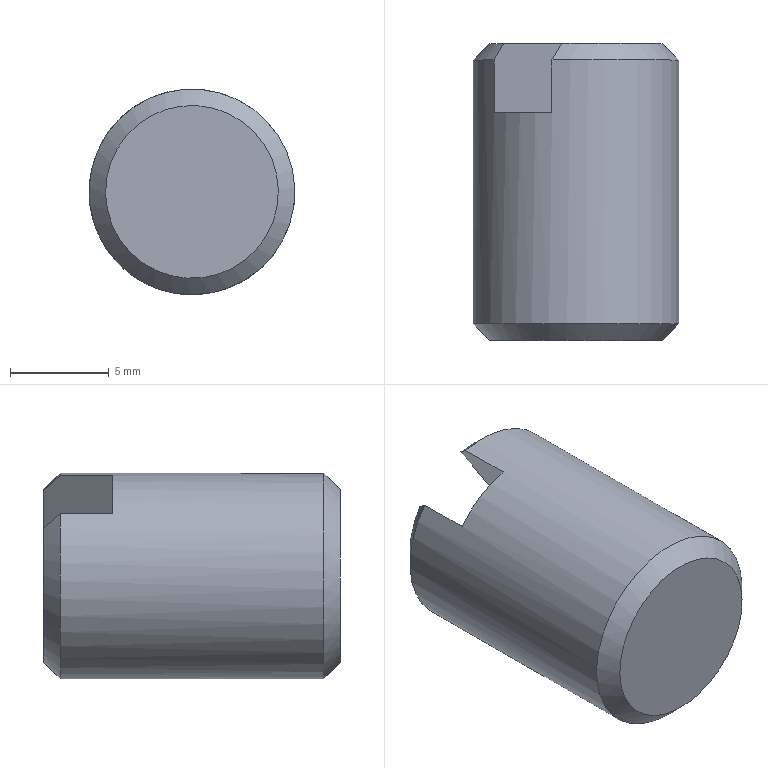Component | NX | 12_PRESSURE_PIN | 1 solid | 10 faces | box 10.4 x 15 x 10.4 mm | volume 1129 mm3 | plane 6 | cone 3 | cylinder 1 | commonest cylinder face diameters 10.396 x1
STEP:
#1=CARTESIAN_POINT('',(0.,0.,0.));
#2=DIRECTION('',(0.,0.,1.));
#3=DIRECTION('',(1.,0.,0.));
#4=AXIS2_PLACEMENT_3D('',#1,#2,#3);
#5=CARTESIAN_POINT('',(-55.431,208.794,-240.61));
#6=VERTEX_POINT('',#5);
#7=CARTESIAN_POINT('',(-59.806,208.794,-233.913));
#8=VERTEX_POINT('',#7);
#9=CARTESIAN_POINT('',(-57.619,208.794,-237.262));
#10=DIRECTION('',(-0.5469,0.,0.8372));
#11=VECTOR('',#10,1.);
#12=LINE('',#9,#11);
#13=CARTESIAN_POINT('',(-59.084,208.794,-238.219));
#14=DIRECTION('',(0.,1.,0.));
#15=DIRECTION('',(0.8372,0.,0.5469));
#16=AXIS2_PLACEMENT_3D('',#13,#14,#15);
#17=PLANE('',#16);
#18=CARTESIAN_POINT('',(1.75,0.));
#19=DIRECTION('',(0.,-1.));
#20=VECTOR('',#19,1.);
#21=LINE('',#18,#20);
#22=(GEOMETRIC_REPRESENTATION_CONTEXT(2)PARAMETRIC_REPRESENTATION_CONTEXT()REPRESENTATION_CONTEXT('',''));
#23=DEFINITIONAL_REPRESENTATION('',(#21),#22);
#24=PCURVE('',#17,#23);
#25=CARTESIAN_POINT('',(-54.337,205.294,-242.285));
#26=DIRECTION('',(-0.8372,0.,-0.5469));
#27=DIRECTION('',(-0.5469,0.,0.8372));
#28=AXIS2_PLACEMENT_3D('',#25,#26,#27);
#29=PLANE('',#28);
#30=CARTESIAN_POINT('',(6.,3.5));
#31=DIRECTION('',(1.,0.));
#32=VECTOR('',#31,1.);
#33=LINE('',#30,#32);
#34=(GEOMETRIC_REPRESENTATION_CONTEXT(2)PARAMETRIC_REPRESENTATION_CONTEXT()REPRESENTATION_CONTEXT('',''));
#35=DEFINITIONAL_REPRESENTATION('',(#33),#34);
#36=PCURVE('',#29,#35);
#37=SURFACE_CURVE('',#12,(#24,#36),.PCURVE_S1.);
#38=EDGE_CURVE('',#6,#8,#37,.T.);
#39=ORIENTED_EDGE('',*,*,#38,.T.);
#40=CARTESIAN_POINT('',(-59.084,208.794,-238.219));
#41=DIRECTION('',(0.,1.,0.));
#42=DIRECTION('',(0.8372,0.,0.5469));
#43=AXIS2_PLACEMENT_3D('',#40,#41,#42);
#44=CIRCLE('',#43,4.366);
#45=CARTESIAN_POINT('',(0.,0.));
#46=DIRECTION('',(1.,-0.));
#47=AXIS2_PLACEMENT_2D('',#45,#46);
#48=CIRCLE('',#47,4.366);
#49=(GEOMETRIC_REPRESENTATION_CONTEXT(2)PARAMETRIC_REPRESENTATION_CONTEXT()REPRESENTATION_CONTEXT('',''));
#50=DEFINITIONAL_REPRESENTATION('',(#48),#49);
#51=PCURVE('',#17,#50);
#52=CARTESIAN_POINT('',(-59.084,207.727,-238.219));
#53=DIRECTION('',(0.,-1.,0.));
#54=DIRECTION('',(-0.8372,0.,-0.5469));
#55=AXIS2_PLACEMENT_3D('',#52,#53,#54);
#56=CONICAL_SURFACE('',#55,5.433,0.7854);
#57=CARTESIAN_POINT('',(9.425,-1.067));
#58=DIRECTION('',(-1.,0.));
#59=VECTOR('',#58,1.);
#60=LINE('',#57,#59);
#61=(GEOMETRIC_REPRESENTATION_CONTEXT(2)PARAMETRIC_REPRESENTATION_CONTEXT()REPRESENTATION_CONTEXT('',''));
#62=DEFINITIONAL_REPRESENTATION('',(#60),#61);
#63=PCURVE('',#56,#62);
#64=SURFACE_CURVE('',#44,(#51,#63),.PCURVE_S1.);
#65=EDGE_CURVE('',#8,#6,#64,.T.);
#66=ORIENTED_EDGE('',*,*,#65,.T.);
#67=EDGE_LOOP('',(#39,#66));
#68=FACE_BOUND('',#67,.T.);
#69=ADVANCED_FACE('',(#68),#17,.T.);
#70=CARTESIAN_POINT('',(-58.361,208.794,-242.525));
#71=VERTEX_POINT('',#70);
#72=CARTESIAN_POINT('',(-62.736,208.794,-235.828));
#73=VERTEX_POINT('',#72);
#74=CARTESIAN_POINT('',(-60.549,208.794,-239.176));
#75=DIRECTION('',(-0.5469,0.,0.8372));
#76=VECTOR('',#75,1.);
#77=LINE('',#74,#76);
#78=CARTESIAN_POINT('',(-59.084,208.794,-238.219));
#79=DIRECTION('',(0.,1.,0.));
#80=DIRECTION('',(0.8372,0.,0.5469));
#81=AXIS2_PLACEMENT_3D('',#78,#79,#80);
#82=PLANE('',#81);
#83=CARTESIAN_POINT('',(-1.75,0.));
#84=DIRECTION('',(0.,-1.));
#85=VECTOR('',#84,1.);
#86=LINE('',#83,#85);
#87=(GEOMETRIC_REPRESENTATION_CONTEXT(2)PARAMETRIC_REPRESENTATION_CONTEXT()REPRESENTATION_CONTEXT('',''));
#88=DEFINITIONAL_REPRESENTATION('',(#86),#87);
#89=PCURVE('',#82,#88);
#90=CARTESIAN_POINT('',(-57.267,205.294,-244.199));
#91=DIRECTION('',(-0.8372,0.,-0.5469));
#92=DIRECTION('',(-0.5469,0.,0.8372));
#93=AXIS2_PLACEMENT_3D('',#90,#91,#92);
#94=PLANE('',#93);
#95=CARTESIAN_POINT('',(6.,3.5));
#96=DIRECTION('',(1.,0.));
#97=VECTOR('',#96,1.);
#98=LINE('',#95,#97);
#99=(GEOMETRIC_REPRESENTATION_CONTEXT(2)PARAMETRIC_REPRESENTATION_CONTEXT()REPRESENTATION_CONTEXT('',''));
#100=DEFINITIONAL_REPRESENTATION('',(#98),#99);
#101=PCURVE('',#94,#100);
#102=SURFACE_CURVE('',#77,(#89,#101),.PCURVE_S1.);
#103=EDGE_CURVE('',#71,#73,#102,.T.);
#104=ORIENTED_EDGE('',*,*,#103,.F.);
#105=CARTESIAN_POINT('',(-59.084,208.794,-238.219));
#106=DIRECTION('',(0.,1.,0.));
#107=DIRECTION('',(0.8372,0.,0.5469));
#108=AXIS2_PLACEMENT_3D('',#105,#106,#107);
#109=CIRCLE('',#108,4.366);
#110=CARTESIAN_POINT('',(0.,0.));
#111=DIRECTION('',(1.,-0.));
#112=AXIS2_PLACEMENT_2D('',#110,#111);
#113=CIRCLE('',#112,4.366);
#114=(GEOMETRIC_REPRESENTATION_CONTEXT(2)PARAMETRIC_REPRESENTATION_CONTEXT()REPRESENTATION_CONTEXT('',''));
#115=DEFINITIONAL_REPRESENTATION('',(#113),#114);
#116=PCURVE('',#82,#115);
#117=CARTESIAN_POINT('',(-59.084,207.727,-238.219));
#118=DIRECTION('',(0.,-1.,0.));
#119=DIRECTION('',(-0.8372,0.,-0.5469));
#120=AXIS2_PLACEMENT_3D('',#117,#118,#119);
#121=CONICAL_SURFACE('',#120,5.433,0.7854);
#122=CARTESIAN_POINT('',(3.142,-1.067));
#123=DIRECTION('',(-1.,-0.));
#124=VECTOR('',#123,1.);
#125=LINE('',#122,#124);
#126=(GEOMETRIC_REPRESENTATION_CONTEXT(2)PARAMETRIC_REPRESENTATION_CONTEXT()REPRESENTATION_CONTEXT('',''));
#127=DEFINITIONAL_REPRESENTATION('',(#125),#126);
#128=PCURVE('',#121,#127);
#129=SURFACE_CURVE('',#109,(#116,#128),.PCURVE_S1.);
#130=EDGE_CURVE('',#71,#73,#129,.T.);
#131=ORIENTED_EDGE('',*,*,#130,.T.);
#132=EDGE_LOOP('',(#104,#131));
#133=FACE_BOUND('',#132,.T.);
#134=ADVANCED_FACE('',(#133),#82,.T.);
#135=CARTESIAN_POINT('',(-62.739,193.794,-240.607));
#136=VERTEX_POINT('',#135);
#137=CARTESIAN_POINT('',(-55.429,193.794,-235.831));
#138=VERTEX_POINT('',#137);
#139=CARTESIAN_POINT('',(-59.084,193.794,-238.219));
#140=DIRECTION('',(0.,-1.,0.));
#141=DIRECTION('',(-0.8372,0.,-0.5469));
#142=AXIS2_PLACEMENT_3D('',#139,#140,#141);
#143=CIRCLE('',#142,4.366);
#144=CARTESIAN_POINT('',(-59.084,193.794,-238.219));
#145=DIRECTION('',(0.,-1.,0.));
#146=DIRECTION('',(-0.8372,0.,-0.5469));
#147=AXIS2_PLACEMENT_3D('',#144,#145,#146);
#148=PLANE('',#147);
#149=CARTESIAN_POINT('',(0.,0.));
#150=DIRECTION('',(1.,0.));
#151=AXIS2_PLACEMENT_2D('',#149,#150);
#152=CIRCLE('',#151,4.366);
#153=(GEOMETRIC_REPRESENTATION_CONTEXT(2)PARAMETRIC_REPRESENTATION_CONTEXT()REPRESENTATION_CONTEXT('',''));
#154=DEFINITIONAL_REPRESENTATION('',(#152),#153);
#155=PCURVE('',#148,#154);
#156=CARTESIAN_POINT('',(-59.084,194.861,-238.219));
#157=DIRECTION('',(0.,1.,0.));
#158=DIRECTION('',(0.8372,0.,0.5469));
#159=AXIS2_PLACEMENT_3D('',#156,#157,#158);
#160=CONICAL_SURFACE('',#159,5.433,0.7854);
#161=CARTESIAN_POINT('',(3.142,-1.067));
#162=DIRECTION('',(-1.,0.));
#163=VECTOR('',#162,1.);
#164=LINE('',#161,#163);
#165=(GEOMETRIC_REPRESENTATION_CONTEXT(2)PARAMETRIC_REPRESENTATION_CONTEXT()REPRESENTATION_CONTEXT('',''));
#166=DEFINITIONAL_REPRESENTATION('',(#164),#165);
#167=PCURVE('',#160,#166);
#168=SURFACE_CURVE('',#143,(#155,#167),.PCURVE_S1.);
#169=EDGE_CURVE('',#136,#138,#168,.T.);
#170=ORIENTED_EDGE('',*,*,#169,.T.);
#171=CARTESIAN_POINT('',(-59.084,193.794,-238.219));
#172=DIRECTION('',(0.,-1.,0.));
#173=DIRECTION('',(-0.8372,0.,-0.5469));
#174=AXIS2_PLACEMENT_3D('',#171,#172,#173);
#175=CIRCLE('',#174,4.366);
#176=CARTESIAN_POINT('',(0.,0.));
#177=DIRECTION('',(1.,0.));
#178=AXIS2_PLACEMENT_2D('',#176,#177);
#179=CIRCLE('',#178,4.366);
#180=(GEOMETRIC_REPRESENTATION_CONTEXT(2)PARAMETRIC_REPRESENTATION_CONTEXT()REPRESENTATION_CONTEXT('',''));
#181=DEFINITIONAL_REPRESENTATION('',(#179),#180);
#182=PCURVE('',#148,#181);
#183=CARTESIAN_POINT('',(9.425,-1.067));
#184=DIRECTION('',(-1.,0.));
#185=VECTOR('',#184,1.);
#186=LINE('',#183,#185);
#187=(GEOMETRIC_REPRESENTATION_CONTEXT(2)PARAMETRIC_REPRESENTATION_CONTEXT()REPRESENTATION_CONTEXT('',''));
#188=DEFINITIONAL_REPRESENTATION('',(#186),#187);
#189=PCURVE('',#160,#188);
#190=SURFACE_CURVE('',#175,(#182,#189),.PCURVE_S1.);
#191=EDGE_CURVE('',#138,#136,#190,.T.);
#192=ORIENTED_EDGE('',*,*,#191,.T.);
#193=EDGE_LOOP('',(#170,#192));
#194=FACE_BOUND('',#193,.T.);
#195=ADVANCED_FACE('',(#194),#148,.T.);
#196=CARTESIAN_POINT('',(-54.732,194.626,-235.376));
#197=VERTEX_POINT('',#196);
#198=CARTESIAN_POINT('',(-59.084,194.626,-238.219));
#199=DIRECTION('',(0.,1.,0.));
#200=DIRECTION('',(0.8372,0.,0.5469));
#201=AXIS2_PLACEMENT_3D('',#198,#199,#200);
#202=CIRCLE('',#201,5.198);
#203=CARTESIAN_POINT('',(-59.084,193.794,-238.219));
#204=DIRECTION('',(0.,1.,0.));
#205=DIRECTION('',(0.8372,0.,0.5469));
#206=AXIS2_PLACEMENT_3D('',#203,#204,#205);
#207=CYLINDRICAL_SURFACE('',#206,5.198);
#208=CARTESIAN_POINT('',(0.,0.8322));
#209=DIRECTION('',(1.,0.));
#210=VECTOR('',#209,1.);
#211=LINE('',#208,#210);
#212=(GEOMETRIC_REPRESENTATION_CONTEXT(2)PARAMETRIC_REPRESENTATION_CONTEXT()REPRESENTATION_CONTEXT('',''));
#213=DEFINITIONAL_REPRESENTATION('',(#211),#212);
#214=PCURVE('',#207,#213);
#215=CARTESIAN_POINT('',(0.,-0.2349));
#216=DIRECTION('',(1.,0.));
#217=VECTOR('',#216,1.);
#218=LINE('',#215,#217);
#219=(GEOMETRIC_REPRESENTATION_CONTEXT(2)PARAMETRIC_REPRESENTATION_CONTEXT()REPRESENTATION_CONTEXT('',''));
#220=DEFINITIONAL_REPRESENTATION('',(#218),#219);
#221=PCURVE('',#160,#220);
#222=SURFACE_CURVE('',#202,(#214,#221),.PCURVE_S1.);
#223=EDGE_CURVE('',#197,#197,#222,.T.);
#224=ORIENTED_EDGE('',*,*,#223,.T.);
#225=CARTESIAN_POINT('',(-54.732,207.961,-235.376));
#226=VERTEX_POINT('',#225);
#227=CARTESIAN_POINT('',(-54.732,194.626,-235.376));
#228=CARTESIAN_POINT('',(-54.732,207.961,-235.376));
#229=B_SPLINE_CURVE_WITH_KNOTS('',1,(#227,#228),.UNSPECIFIED.,.F.,.F.,(2,2),(0.8322,14.168),.PIECEWISE_BEZIER_KNOTS.);
#230=CARTESIAN_POINT('',(6.283,0.));
#231=DIRECTION('',(0.,1.));
#232=VECTOR('',#231,1.);
#233=LINE('',#230,#232);
#234=(GEOMETRIC_REPRESENTATION_CONTEXT(2)PARAMETRIC_REPRESENTATION_CONTEXT()REPRESENTATION_CONTEXT('',''));
#235=DEFINITIONAL_REPRESENTATION('',(#233),#234);
#236=PCURVE('',#207,#235);
#237=CARTESIAN_POINT('',(0.,0.));
#238=DIRECTION('',(0.,1.));
#239=VECTOR('',#238,1.);
#240=LINE('',#237,#239);
#241=(GEOMETRIC_REPRESENTATION_CONTEXT(2)PARAMETRIC_REPRESENTATION_CONTEXT()REPRESENTATION_CONTEXT('',''));
#242=DEFINITIONAL_REPRESENTATION('',(#240),#241);
#243=PCURVE('',#207,#242);
#244=SEAM_CURVE('',#229,(#236,#243),.PCURVE_S1.);
#245=EDGE_CURVE('',#197,#226,#244,.T.);
#246=ORIENTED_EDGE('',*,*,#245,.T.);
#247=CARTESIAN_POINT('',(-60.296,207.961,-233.164));
#248=VERTEX_POINT('',#247);
#249=CARTESIAN_POINT('',(-59.084,207.961,-238.219));
#250=DIRECTION('',(0.,-1.,0.));
#251=DIRECTION('',(-0.8372,0.,-0.5469));
#252=AXIS2_PLACEMENT_3D('',#249,#250,#251);
#253=CIRCLE('',#252,5.198);
#254=CARTESIAN_POINT('',(9.425,14.168));
#255=DIRECTION('',(-1.,0.));
#256=VECTOR('',#255,1.);
#257=LINE('',#254,#256);
#258=(GEOMETRIC_REPRESENTATION_CONTEXT(2)PARAMETRIC_REPRESENTATION_CONTEXT()REPRESENTATION_CONTEXT('',''));
#259=DEFINITIONAL_REPRESENTATION('',(#257),#258);
#260=PCURVE('',#207,#259);
#261=CARTESIAN_POINT('',(-0.,-0.2349));
#262=DIRECTION('',(1.,-0.));
#263=VECTOR('',#262,1.);
#264=LINE('',#261,#263);
#265=(GEOMETRIC_REPRESENTATION_CONTEXT(2)PARAMETRIC_REPRESENTATION_CONTEXT()REPRESENTATION_CONTEXT('',''));
#266=DEFINITIONAL_REPRESENTATION('',(#264),#265);
#267=PCURVE('',#56,#266);
#268=SURFACE_CURVE('',#253,(#260,#267),.PCURVE_S1.);
#269=EDGE_CURVE('',#226,#248,#268,.T.);
#270=ORIENTED_EDGE('',*,*,#269,.T.);
#271=CARTESIAN_POINT('',(-60.296,205.294,-233.164));
#272=VERTEX_POINT('',#271);
#273=CARTESIAN_POINT('',(-60.296,207.961,-233.164));
#274=DIRECTION('',(0.,-1.,0.));
#275=VECTOR('',#274,1.);
#276=LINE('',#273,#275);
#277=CARTESIAN_POINT('',(5.056,14.168));
#278=DIRECTION('',(0.,-1.));
#279=VECTOR('',#278,1.);
#280=LINE('',#277,#279);
#281=(GEOMETRIC_REPRESENTATION_CONTEXT(2)PARAMETRIC_REPRESENTATION_CONTEXT()REPRESENTATION_CONTEXT('',''));
#282=DEFINITIONAL_REPRESENTATION('',(#280),#281);
#283=PCURVE('',#207,#282);
#284=CARTESIAN_POINT('',(10.895,2.668));
#285=DIRECTION('',(0.,-1.));
#286=VECTOR('',#285,1.);
#287=LINE('',#284,#286);
#288=(GEOMETRIC_REPRESENTATION_CONTEXT(2)PARAMETRIC_REPRESENTATION_CONTEXT()REPRESENTATION_CONTEXT('',''));
#289=DEFINITIONAL_REPRESENTATION('',(#287),#288);
#290=PCURVE('',#29,#289);
#291=SURFACE_CURVE('',#276,(#283,#290),.PCURVE_S1.);
#292=EDGE_CURVE('',#248,#272,#291,.T.);
#293=ORIENTED_EDGE('',*,*,#292,.T.);
#294=CARTESIAN_POINT('',(-63.226,205.294,-235.079));
#295=VERTEX_POINT('',#294);
#296=CARTESIAN_POINT('',(-59.084,205.294,-238.219));
#297=DIRECTION('',(0.,1.,0.));
#298=DIRECTION('',(-0.8372,0.,-0.5469));
#299=AXIS2_PLACEMENT_3D('',#296,#297,#298);
#300=CIRCLE('',#299,5.198);
#301=CARTESIAN_POINT('',(3.142,11.5));
#302=DIRECTION('',(1.,0.));
#303=VECTOR('',#302,1.);
#304=LINE('',#301,#303);
#305=(GEOMETRIC_REPRESENTATION_CONTEXT(2)PARAMETRIC_REPRESENTATION_CONTEXT()REPRESENTATION_CONTEXT('',''));
#306=DEFINITIONAL_REPRESENTATION('',(#304),#305);
#307=PCURVE('',#207,#306);
#308=CARTESIAN_POINT('',(-55.802,205.294,-243.242));
#309=DIRECTION('',(0.,-1.,0.));
#310=DIRECTION('',(-0.5469,0.,0.8372));
#311=AXIS2_PLACEMENT_3D('',#308,#309,#310);
#312=PLANE('',#311);
#313=CARTESIAN_POINT('',(6.,5.198));
#314=CARTESIAN_POINT('',(15.003,5.198));
#315=CARTESIAN_POINT('',(10.502,-2.599));
#316=CARTESIAN_POINT('',(6.,-10.396));
#317=CARTESIAN_POINT('',(1.498,-2.599));
#318=CARTESIAN_POINT('',(-3.003,5.198));
#319=CARTESIAN_POINT('',(6.,5.198));
#320=(BOUNDED_CURVE()B_SPLINE_CURVE(2,(#313,#314,#315,#316,#317,#318,#319),.UNSPECIFIED.,.T.,.F.)B_SPLINE_CURVE_WITH_KNOTS((1,2,2,2,2,1),(-2.094,0.,2.094,4.189,6.283,8.378),.UNSPECIFIED.)CURVE()GEOMETRIC_REPRESENTATION_ITEM()RATIONAL_B_SPLINE_CURVE((1.,0.5,1.,0.5,1.,0.5,1.))REPRESENTATION_ITEM(''));
#321=(GEOMETRIC_REPRESENTATION_CONTEXT(2)PARAMETRIC_REPRESENTATION_CONTEXT()REPRESENTATION_CONTEXT('',''));
#322=DEFINITIONAL_REPRESENTATION('',(#320),#321);
#323=PCURVE('',#312,#322);
#324=SURFACE_CURVE('',#300,(#307,#323),.PCURVE_S1.);
#325=EDGE_CURVE('',#295,#272,#324,.T.);
#326=ORIENTED_EDGE('',*,*,#325,.F.);
#327=CARTESIAN_POINT('',(-63.226,207.961,-235.079));
#328=VERTEX_POINT('',#327);
#329=CARTESIAN_POINT('',(-63.226,193.794,-235.079));
#330=DIRECTION('',(0.,-1.,0.));
#331=VECTOR('',#330,1.);
#332=LINE('',#329,#331);
#333=CARTESIAN_POINT('',(4.369,0.));
#334=DIRECTION('',(0.,-1.));
#335=VECTOR('',#334,1.);
#336=LINE('',#333,#335);
#337=(GEOMETRIC_REPRESENTATION_CONTEXT(2)PARAMETRIC_REPRESENTATION_CONTEXT()REPRESENTATION_CONTEXT('',''));
#338=DEFINITIONAL_REPRESENTATION('',(#336),#337);
#339=PCURVE('',#207,#338);
#340=CARTESIAN_POINT('',(10.895,-11.5));
#341=DIRECTION('',(0.,-1.));
#342=VECTOR('',#341,1.);
#343=LINE('',#340,#342);
#344=(GEOMETRIC_REPRESENTATION_CONTEXT(2)PARAMETRIC_REPRESENTATION_CONTEXT()REPRESENTATION_CONTEXT('',''));
#345=DEFINITIONAL_REPRESENTATION('',(#343),#344);
#346=PCURVE('',#94,#345);
#347=SURFACE_CURVE('',#332,(#339,#346),.PCURVE_S1.);
#348=EDGE_CURVE('',#328,#295,#347,.T.);
#349=ORIENTED_EDGE('',*,*,#348,.F.);
#350=CARTESIAN_POINT('',(-57.872,207.961,-243.274));
#351=VERTEX_POINT('',#350);
#352=CARTESIAN_POINT('',(-59.084,207.961,-238.219));
#353=DIRECTION('',(0.,-1.,0.));
#354=DIRECTION('',(-0.8372,0.,-0.5469));
#355=AXIS2_PLACEMENT_3D('',#352,#353,#354);
#356=CIRCLE('',#355,5.198);
#357=CARTESIAN_POINT('',(9.425,14.168));
#358=DIRECTION('',(-1.,0.));
#359=VECTOR('',#358,1.);
#360=LINE('',#357,#359);
#361=(GEOMETRIC_REPRESENTATION_CONTEXT(2)PARAMETRIC_REPRESENTATION_CONTEXT()REPRESENTATION_CONTEXT('',''));
#362=DEFINITIONAL_REPRESENTATION('',(#360),#361);
#363=PCURVE('',#207,#362);
#364=CARTESIAN_POINT('',(-6.283,-0.2349));
#365=DIRECTION('',(1.,0.));
#366=VECTOR('',#365,1.);
#367=LINE('',#364,#366);
#368=(GEOMETRIC_REPRESENTATION_CONTEXT(2)PARAMETRIC_REPRESENTATION_CONTEXT()REPRESENTATION_CONTEXT('',''));
#369=DEFINITIONAL_REPRESENTATION('',(#367),#368);
#370=PCURVE('',#121,#369);
#371=SURFACE_CURVE('',#356,(#363,#370),.PCURVE_S1.);
#372=EDGE_CURVE('',#328,#351,#371,.T.);
#373=ORIENTED_EDGE('',*,*,#372,.T.);
#374=CARTESIAN_POINT('',(-57.872,205.294,-243.274));
#375=VERTEX_POINT('',#374);
#376=CARTESIAN_POINT('',(-57.872,205.294,-243.274));
#377=DIRECTION('',(0.,1.,0.));
#378=VECTOR('',#377,1.);
#379=LINE('',#376,#378);
#380=CARTESIAN_POINT('',(1.914,11.5));
#381=DIRECTION('',(0.,1.));
#382=VECTOR('',#381,1.);
#383=LINE('',#380,#382);
#384=(GEOMETRIC_REPRESENTATION_CONTEXT(2)PARAMETRIC_REPRESENTATION_CONTEXT()REPRESENTATION_CONTEXT('',''));
#385=DEFINITIONAL_REPRESENTATION('',(#383),#384);
#386=PCURVE('',#207,#385);
#387=CARTESIAN_POINT('',(1.105,0.));
#388=DIRECTION('',(0.,1.));
#389=VECTOR('',#388,1.);
#390=LINE('',#387,#389);
#391=(GEOMETRIC_REPRESENTATION_CONTEXT(2)PARAMETRIC_REPRESENTATION_CONTEXT()REPRESENTATION_CONTEXT('',''));
#392=DEFINITIONAL_REPRESENTATION('',(#390),#391);
#393=PCURVE('',#94,#392);
#394=SURFACE_CURVE('',#379,(#386,#393),.PCURVE_S1.);
#395=EDGE_CURVE('',#375,#351,#394,.T.);
#396=ORIENTED_EDGE('',*,*,#395,.F.);
#397=CARTESIAN_POINT('',(-54.942,205.294,-241.359));
#398=VERTEX_POINT('',#397);
#399=CARTESIAN_POINT('',(-59.084,205.294,-238.219));
#400=DIRECTION('',(0.,1.,0.));
#401=DIRECTION('',(-0.8372,0.,-0.5469));
#402=AXIS2_PLACEMENT_3D('',#399,#400,#401);
#403=CIRCLE('',#402,5.198);
#404=CARTESIAN_POINT('',(-3.142,11.5));
#405=DIRECTION('',(1.,0.));
#406=VECTOR('',#405,1.);
#407=LINE('',#404,#406);
#408=(GEOMETRIC_REPRESENTATION_CONTEXT(2)PARAMETRIC_REPRESENTATION_CONTEXT()REPRESENTATION_CONTEXT('',''));
#409=DEFINITIONAL_REPRESENTATION('',(#407),#408);
#410=PCURVE('',#207,#409);
#411=CARTESIAN_POINT('',(6.,5.198));
#412=CARTESIAN_POINT('',(15.003,5.198));
#413=CARTESIAN_POINT('',(10.502,-2.599));
#414=CARTESIAN_POINT('',(6.,-10.396));
#415=CARTESIAN_POINT('',(1.498,-2.599));
#416=CARTESIAN_POINT('',(-3.003,5.198));
#417=CARTESIAN_POINT('',(6.,5.198));
#418=(BOUNDED_CURVE()B_SPLINE_CURVE(2,(#411,#412,#413,#414,#415,#416,#417),.UNSPECIFIED.,.T.,.F.)B_SPLINE_CURVE_WITH_KNOTS((1,2,2,2,2,1),(-2.094,0.,2.094,4.189,6.283,8.378),.UNSPECIFIED.)CURVE()GEOMETRIC_REPRESENTATION_ITEM()RATIONAL_B_SPLINE_CURVE((1.,0.5,1.,0.5,1.,0.5,1.))REPRESENTATION_ITEM(''));
#419=(GEOMETRIC_REPRESENTATION_CONTEXT(2)PARAMETRIC_REPRESENTATION_CONTEXT()REPRESENTATION_CONTEXT('',''));
#420=DEFINITIONAL_REPRESENTATION('',(#418),#419);
#421=PCURVE('',#312,#420);
#422=SURFACE_CURVE('',#403,(#410,#421),.PCURVE_S1.);
#423=EDGE_CURVE('',#398,#375,#422,.T.);
#424=ORIENTED_EDGE('',*,*,#423,.F.);
#425=CARTESIAN_POINT('',(-54.942,207.961,-241.359));
#426=VERTEX_POINT('',#425);
#427=CARTESIAN_POINT('',(-54.942,193.794,-241.359));
#428=DIRECTION('',(0.,1.,0.));
#429=VECTOR('',#428,1.);
#430=LINE('',#427,#429);
#431=CARTESIAN_POINT('',(1.227,0.));
#432=DIRECTION('',(0.,1.));
#433=VECTOR('',#432,1.);
#434=LINE('',#431,#433);
#435=(GEOMETRIC_REPRESENTATION_CONTEXT(2)PARAMETRIC_REPRESENTATION_CONTEXT()REPRESENTATION_CONTEXT('',''));
#436=DEFINITIONAL_REPRESENTATION('',(#434),#435);
#437=PCURVE('',#207,#436);
#438=CARTESIAN_POINT('',(1.105,-11.5));
#439=DIRECTION('',(0.,1.));
#440=VECTOR('',#439,1.);
#441=LINE('',#438,#440);
#442=(GEOMETRIC_REPRESENTATION_CONTEXT(2)PARAMETRIC_REPRESENTATION_CONTEXT()REPRESENTATION_CONTEXT('',''));
#443=DEFINITIONAL_REPRESENTATION('',(#441),#442);
#444=PCURVE('',#29,#443);
#445=SURFACE_CURVE('',#430,(#437,#444),.PCURVE_S1.);
#446=EDGE_CURVE('',#398,#426,#445,.T.);
#447=ORIENTED_EDGE('',*,*,#446,.T.);
#448=CARTESIAN_POINT('',(-59.084,207.961,-238.219));
#449=DIRECTION('',(0.,-1.,0.));
#450=DIRECTION('',(-0.8372,0.,-0.5469));
#451=AXIS2_PLACEMENT_3D('',#448,#449,#450);
#452=CIRCLE('',#451,5.198);
#453=CARTESIAN_POINT('',(3.142,14.168));
#454=DIRECTION('',(-1.,0.));
#455=VECTOR('',#454,1.);
#456=LINE('',#453,#455);
#457=(GEOMETRIC_REPRESENTATION_CONTEXT(2)PARAMETRIC_REPRESENTATION_CONTEXT()REPRESENTATION_CONTEXT('',''));
#458=DEFINITIONAL_REPRESENTATION('',(#456),#457);
#459=PCURVE('',#207,#458);
#460=CARTESIAN_POINT('',(-0.,-0.2349));
#461=DIRECTION('',(1.,-0.));
#462=VECTOR('',#461,1.);
#463=LINE('',#460,#462);
#464=(GEOMETRIC_REPRESENTATION_CONTEXT(2)PARAMETRIC_REPRESENTATION_CONTEXT()REPRESENTATION_CONTEXT('',''));
#465=DEFINITIONAL_REPRESENTATION('',(#463),#464);
#466=PCURVE('',#56,#465);
#467=SURFACE_CURVE('',#452,(#459,#466),.PCURVE_S1.);
#468=EDGE_CURVE('',#426,#226,#467,.T.);
#469=ORIENTED_EDGE('',*,*,#468,.T.);
#470=ORIENTED_EDGE('',*,*,#245,.F.);
#471=EDGE_LOOP('',(#224,#246,#270,#293,#326,#349,#373,#396,#424,#447,#469,#470));
#472=FACE_BOUND('',#471,.T.);
#473=ADVANCED_FACE('',(#472),#207,.T.);
#474=CARTESIAN_POINT('',(-57.267,205.294,-244.199));
#475=DIRECTION('',(0.5469,0.,-0.8372));
#476=VECTOR('',#475,1.);
#477=LINE('',#474,#476);
#478=CARTESIAN_POINT('',(0.,1.75));
#479=DIRECTION('',(-1.,0.));
#480=VECTOR('',#479,1.);
#481=LINE('',#478,#480);
#482=(GEOMETRIC_REPRESENTATION_CONTEXT(2)PARAMETRIC_REPRESENTATION_CONTEXT()REPRESENTATION_CONTEXT('',''));
#483=DEFINITIONAL_REPRESENTATION('',(#481),#482);
#484=PCURVE('',#312,#483);
#485=CARTESIAN_POINT('',(0.,0.));
#486=DIRECTION('',(-1.,0.));
#487=VECTOR('',#486,1.);
#488=LINE('',#485,#487);
#489=(GEOMETRIC_REPRESENTATION_CONTEXT(2)PARAMETRIC_REPRESENTATION_CONTEXT()REPRESENTATION_CONTEXT('',''));
#490=DEFINITIONAL_REPRESENTATION('',(#488),#489);
#491=PCURVE('',#94,#490);
#492=SURFACE_CURVE('',#477,(#484,#491),.PCURVE_S1.);
#493=EDGE_CURVE('',#295,#375,#492,.T.);
#494=ORIENTED_EDGE('',*,*,#493,.F.);
#495=ORIENTED_EDGE('',*,*,#325,.T.);
#496=CARTESIAN_POINT('',(-54.337,205.294,-242.285));
#497=DIRECTION('',(0.5469,0.,-0.8372));
#498=VECTOR('',#497,1.);
#499=LINE('',#496,#498);
#500=CARTESIAN_POINT('',(0.,-1.75));
#501=DIRECTION('',(-1.,0.));
#502=VECTOR('',#501,1.);
#503=LINE('',#500,#502);
#504=(GEOMETRIC_REPRESENTATION_CONTEXT(2)PARAMETRIC_REPRESENTATION_CONTEXT()REPRESENTATION_CONTEXT('',''));
#505=DEFINITIONAL_REPRESENTATION('',(#503),#504);
#506=PCURVE('',#312,#505);
#507=CARTESIAN_POINT('',(0.,0.));
#508=DIRECTION('',(-1.,0.));
#509=VECTOR('',#508,1.);
#510=LINE('',#507,#509);
#511=(GEOMETRIC_REPRESENTATION_CONTEXT(2)PARAMETRIC_REPRESENTATION_CONTEXT()REPRESENTATION_CONTEXT('',''));
#512=DEFINITIONAL_REPRESENTATION('',(#510),#511);
#513=PCURVE('',#29,#512);
#514=SURFACE_CURVE('',#499,(#506,#513),.PCURVE_S1.);
#515=EDGE_CURVE('',#272,#398,#514,.T.);
#516=ORIENTED_EDGE('',*,*,#515,.T.);
#517=ORIENTED_EDGE('',*,*,#423,.T.);
#518=EDGE_LOOP('',(#494,#495,#516,#517));
#519=FACE_BOUND('',#518,.T.);
#520=ADVANCED_FACE('',(#519),#312,.F.);
#521=ORIENTED_EDGE('',*,*,#395,.T.);
#522=CARTESIAN_POINT('',(-57.872,207.961,-243.274));
#523=CARTESIAN_POINT('',(-58.034,208.241,-243.026));
#524=CARTESIAN_POINT('',(-58.197,208.518,-242.776));
#525=CARTESIAN_POINT('',(-58.361,208.794,-242.525));
#526=B_SPLINE_CURVE_WITH_KNOTS('',3,(#522,#523,#524,#525),.UNSPECIFIED.,.F.,.F.,(4,4),(0.,1.),.PIECEWISE_BEZIER_KNOTS.);
#527=CARTESIAN_POINT('',(1.105,2.668));
#528=CARTESIAN_POINT('',(1.402,2.947));
#529=CARTESIAN_POINT('',(1.7,3.225));
#530=CARTESIAN_POINT('',(2.,3.5));
#531=B_SPLINE_CURVE_WITH_KNOTS('',3,(#527,#528,#529,#530),.UNSPECIFIED.,.F.,.F.,(4,4),(0.,1.),.PIECEWISE_BEZIER_KNOTS.);
#532=(GEOMETRIC_REPRESENTATION_CONTEXT(2)PARAMETRIC_REPRESENTATION_CONTEXT()REPRESENTATION_CONTEXT('',''));
#533=DEFINITIONAL_REPRESENTATION('',(#531),#532);
#534=PCURVE('',#94,#533);
#535=CARTESIAN_POINT('',(1.227,-0.2349));
#536=CARTESIAN_POINT('',(1.158,-1.067));
#537=B_SPLINE_CURVE_WITH_KNOTS('',1,(#535,#536),.UNSPECIFIED.,.F.,.F.,(2,2),(0.,1.),.PIECEWISE_BEZIER_KNOTS.);
#538=(GEOMETRIC_REPRESENTATION_CONTEXT(2)PARAMETRIC_REPRESENTATION_CONTEXT()REPRESENTATION_CONTEXT('',''));
#539=DEFINITIONAL_REPRESENTATION('',(#537),#538);
#540=PCURVE('',#121,#539);
#541=SURFACE_CURVE('',#526,(#534,#540),.PCURVE_S1.);
#542=EDGE_CURVE('',#351,#71,#541,.T.);
#543=ORIENTED_EDGE('',*,*,#542,.T.);
#544=ORIENTED_EDGE('',*,*,#103,.T.);
#545=CARTESIAN_POINT('',(-62.736,208.794,-235.828));
#546=CARTESIAN_POINT('',(-62.901,208.518,-235.576));
#547=CARTESIAN_POINT('',(-63.064,208.241,-235.327));
#548=CARTESIAN_POINT('',(-63.226,207.961,-235.079));
#549=B_SPLINE_CURVE_WITH_KNOTS('',3,(#545,#546,#547,#548),.UNSPECIFIED.,.F.,.F.,(4,4),(0.,1.),.PIECEWISE_BEZIER_KNOTS.);
#550=CARTESIAN_POINT('',(10.,3.5));
#551=CARTESIAN_POINT('',(10.3,3.225));
#552=CARTESIAN_POINT('',(10.598,2.947));
#553=CARTESIAN_POINT('',(10.895,2.668));
#554=B_SPLINE_CURVE_WITH_KNOTS('',3,(#550,#551,#552,#553),.UNSPECIFIED.,.F.,.F.,(4,4),(0.,1.),.PIECEWISE_BEZIER_KNOTS.);
#555=(GEOMETRIC_REPRESENTATION_CONTEXT(2)PARAMETRIC_REPRESENTATION_CONTEXT()REPRESENTATION_CONTEXT('',''));
#556=DEFINITIONAL_REPRESENTATION('',(#554),#555);
#557=PCURVE('',#94,#556);
#558=CARTESIAN_POINT('',(-1.158,-1.067));
#559=CARTESIAN_POINT('',(-1.227,-0.2349));
#560=B_SPLINE_CURVE_WITH_KNOTS('',1,(#558,#559),.UNSPECIFIED.,.F.,.F.,(2,2),(0.,1.),.PIECEWISE_BEZIER_KNOTS.);
#561=(GEOMETRIC_REPRESENTATION_CONTEXT(2)PARAMETRIC_REPRESENTATION_CONTEXT()REPRESENTATION_CONTEXT('',''));
#562=DEFINITIONAL_REPRESENTATION('',(#560),#561);
#563=PCURVE('',#121,#562);
#564=SURFACE_CURVE('',#549,(#557,#563),.PCURVE_S1.);
#565=EDGE_CURVE('',#73,#328,#564,.T.);
#566=ORIENTED_EDGE('',*,*,#565,.T.);
#567=ORIENTED_EDGE('',*,*,#348,.T.);
#568=ORIENTED_EDGE('',*,*,#493,.T.);
#569=EDGE_LOOP('',(#521,#543,#544,#566,#567,#568));
#570=FACE_BOUND('',#569,.T.);
#571=ADVANCED_FACE('',(#570),#94,.F.);
#572=ORIENTED_EDGE('',*,*,#292,.F.);
#573=CARTESIAN_POINT('',(-60.296,207.961,-233.164));
#574=CARTESIAN_POINT('',(-60.134,208.241,-233.413));
#575=CARTESIAN_POINT('',(-59.971,208.518,-233.662));
#576=CARTESIAN_POINT('',(-59.806,208.794,-233.913));
#577=B_SPLINE_CURVE_WITH_KNOTS('',3,(#573,#574,#575,#576),.UNSPECIFIED.,.F.,.F.,(4,4),(0.,1.),.PIECEWISE_BEZIER_KNOTS.);
#578=CARTESIAN_POINT('',(10.895,2.668));
#579=CARTESIAN_POINT('',(10.598,2.947));
#580=CARTESIAN_POINT('',(10.3,3.225));
#581=CARTESIAN_POINT('',(10.,3.5));
#582=B_SPLINE_CURVE_WITH_KNOTS('',3,(#578,#579,#580,#581),.UNSPECIFIED.,.F.,.F.,(4,4),(0.,1.),.PIECEWISE_BEZIER_KNOTS.);
#583=(GEOMETRIC_REPRESENTATION_CONTEXT(2)PARAMETRIC_REPRESENTATION_CONTEXT()REPRESENTATION_CONTEXT('',''));
#584=DEFINITIONAL_REPRESENTATION('',(#582),#583);
#585=PCURVE('',#29,#584);
#586=CARTESIAN_POINT('',(4.369,-0.2349));
#587=CARTESIAN_POINT('',(4.3,-1.067));
#588=B_SPLINE_CURVE_WITH_KNOTS('',1,(#586,#587),.UNSPECIFIED.,.F.,.F.,(2,2),(0.,1.),.PIECEWISE_BEZIER_KNOTS.);
#589=(GEOMETRIC_REPRESENTATION_CONTEXT(2)PARAMETRIC_REPRESENTATION_CONTEXT()REPRESENTATION_CONTEXT('',''));
#590=DEFINITIONAL_REPRESENTATION('',(#588),#589);
#591=PCURVE('',#56,#590);
#592=SURFACE_CURVE('',#577,(#585,#591),.PCURVE_S1.);
#593=EDGE_CURVE('',#248,#8,#592,.T.);
#594=ORIENTED_EDGE('',*,*,#593,.T.);
#595=ORIENTED_EDGE('',*,*,#38,.F.);
#596=CARTESIAN_POINT('',(-55.431,208.794,-240.61));
#597=CARTESIAN_POINT('',(-55.267,208.518,-240.862));
#598=CARTESIAN_POINT('',(-55.104,208.241,-241.111));
#599=CARTESIAN_POINT('',(-54.942,207.961,-241.359));
#600=B_SPLINE_CURVE_WITH_KNOTS('',3,(#596,#597,#598,#599),.UNSPECIFIED.,.F.,.F.,(4,4),(0.,1.),.PIECEWISE_BEZIER_KNOTS.);
#601=CARTESIAN_POINT('',(2.,3.5));
#602=CARTESIAN_POINT('',(1.7,3.225));
#603=CARTESIAN_POINT('',(1.402,2.947));
#604=CARTESIAN_POINT('',(1.105,2.668));
#605=B_SPLINE_CURVE_WITH_KNOTS('',3,(#601,#602,#603,#604),.UNSPECIFIED.,.F.,.F.,(4,4),(0.,1.),.PIECEWISE_BEZIER_KNOTS.);
#606=(GEOMETRIC_REPRESENTATION_CONTEXT(2)PARAMETRIC_REPRESENTATION_CONTEXT()REPRESENTATION_CONTEXT('',''));
#607=DEFINITIONAL_REPRESENTATION('',(#605),#606);
#608=PCURVE('',#29,#607);
#609=CARTESIAN_POINT('',(1.983,-1.067));
#610=CARTESIAN_POINT('',(1.914,-0.2349));
#611=B_SPLINE_CURVE_WITH_KNOTS('',1,(#609,#610),.UNSPECIFIED.,.F.,.F.,(2,2),(0.,1.),.PIECEWISE_BEZIER_KNOTS.);
#612=(GEOMETRIC_REPRESENTATION_CONTEXT(2)PARAMETRIC_REPRESENTATION_CONTEXT()REPRESENTATION_CONTEXT('',''));
#613=DEFINITIONAL_REPRESENTATION('',(#611),#612);
#614=PCURVE('',#56,#613);
#615=SURFACE_CURVE('',#600,(#608,#614),.PCURVE_S1.);
#616=EDGE_CURVE('',#6,#426,#615,.T.);
#617=ORIENTED_EDGE('',*,*,#616,.T.);
#618=ORIENTED_EDGE('',*,*,#446,.F.);
#619=ORIENTED_EDGE('',*,*,#515,.F.);
#620=EDGE_LOOP('',(#572,#594,#595,#617,#618,#619));
#621=FACE_BOUND('',#620,.T.);
#622=ADVANCED_FACE('',(#621),#29,.T.);
#623=ORIENTED_EDGE('',*,*,#191,.F.);
#624=CARTESIAN_POINT('',(-55.429,193.794,-235.831));
#625=CARTESIAN_POINT('',(-54.732,194.626,-235.376));
#626=B_SPLINE_CURVE_WITH_KNOTS('',1,(#624,#625),.UNSPECIFIED.,.F.,.F.,(2,2),(-1.509,-0.3322),.PIECEWISE_BEZIER_KNOTS.);
#627=CARTESIAN_POINT('',(6.283,0.));
#628=DIRECTION('',(0.,1.));
#629=VECTOR('',#628,1.);
#630=LINE('',#627,#629);
#631=(GEOMETRIC_REPRESENTATION_CONTEXT(2)PARAMETRIC_REPRESENTATION_CONTEXT()REPRESENTATION_CONTEXT('',''));
#632=DEFINITIONAL_REPRESENTATION('',(#630),#631);
#633=PCURVE('',#160,#632);
#634=CARTESIAN_POINT('',(0.,0.));
#635=DIRECTION('',(0.,1.));
#636=VECTOR('',#635,1.);
#637=LINE('',#634,#636);
#638=(GEOMETRIC_REPRESENTATION_CONTEXT(2)PARAMETRIC_REPRESENTATION_CONTEXT()REPRESENTATION_CONTEXT('',''));
#639=DEFINITIONAL_REPRESENTATION('',(#637),#638);
#640=PCURVE('',#160,#639);
#641=SEAM_CURVE('',#626,(#633,#640),.PCURVE_S1.);
#642=EDGE_CURVE('',#138,#197,#641,.T.);
#643=ORIENTED_EDGE('',*,*,#642,.T.);
#644=ORIENTED_EDGE('',*,*,#223,.F.);
#645=ORIENTED_EDGE('',*,*,#642,.F.);
#646=ORIENTED_EDGE('',*,*,#169,.F.);
#647=EDGE_LOOP('',(#623,#643,#644,#645,#646));
#648=FACE_BOUND('',#647,.T.);
#649=ADVANCED_FACE('',(#648),#160,.T.);
#650=ORIENTED_EDGE('',*,*,#616,.F.);
#651=ORIENTED_EDGE('',*,*,#65,.F.);
#652=ORIENTED_EDGE('',*,*,#593,.F.);
#653=ORIENTED_EDGE('',*,*,#269,.F.);
#654=ORIENTED_EDGE('',*,*,#468,.F.);
#655=EDGE_LOOP('',(#650,#651,#652,#653,#654));
#656=FACE_BOUND('',#655,.T.);
#657=ADVANCED_FACE('',(#656),#56,.T.);
#658=ORIENTED_EDGE('',*,*,#565,.F.);
#659=ORIENTED_EDGE('',*,*,#130,.F.);
#660=ORIENTED_EDGE('',*,*,#542,.F.);
#661=ORIENTED_EDGE('',*,*,#372,.F.);
#662=EDGE_LOOP('',(#658,#659,#660,#661));
#663=FACE_BOUND('',#662,.T.);
#664=ADVANCED_FACE('',(#663),#121,.T.);
#665=CLOSED_SHELL('',(#69,#134,#195,#473,#520,#571,#622,#649,#657,#664));
#666=MANIFOLD_SOLID_BREP('',#665);
#667=(LENGTH_UNIT()NAMED_UNIT(*)SI_UNIT(.MILLI.,.METRE.));
#668=UNCERTAINTY_MEASURE_WITH_UNIT(LENGTH_MEASURE(0.005),#667,'','');
#669=(NAMED_UNIT(*)PLANE_ANGLE_UNIT()SI_UNIT($,.RADIAN.));
#670=(NAMED_UNIT(*)SI_UNIT($,.STERADIAN.)SOLID_ANGLE_UNIT());
#671=(GEOMETRIC_REPRESENTATION_CONTEXT(3)GLOBAL_UNCERTAINTY_ASSIGNED_CONTEXT((#668))GLOBAL_UNIT_ASSIGNED_CONTEXT((#667,#669,#670))REPRESENTATION_CONTEXT('',''));
#672=ADVANCED_BREP_SHAPE_REPRESENTATION('',(#4,#666),#671);